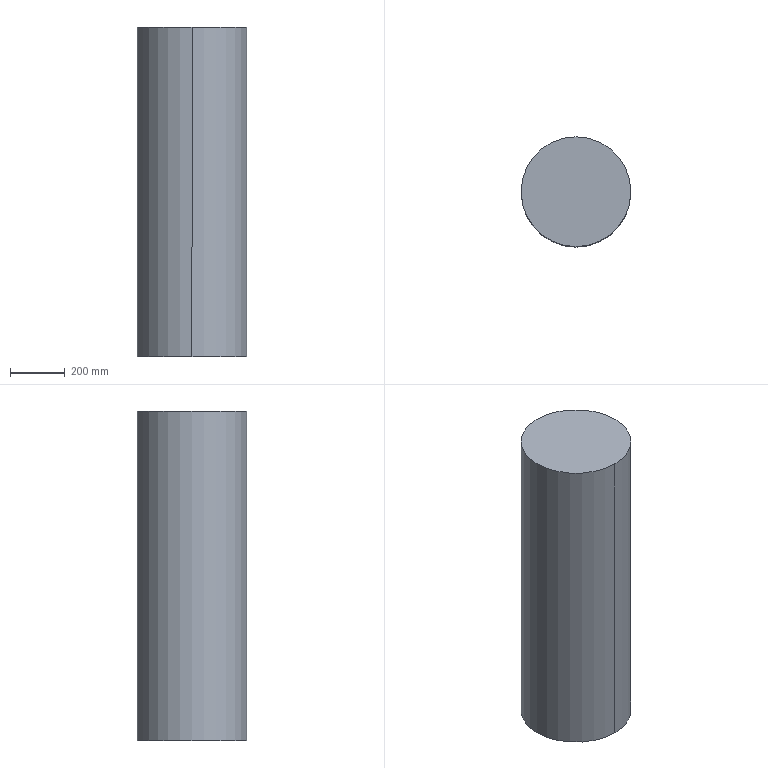Component | SolidWorks | FlexibleLegPinAxis-1 | 1 solid | 4 faces | box 400 x 400 x 1200 mm | volume 150796447 mm3 | cylinder 2 | plane 2 | commonest cylinder face diameters 400 x2
build123d program:
from build123d import *

# Parameters (mm, degrees)
SKETCH1_R           = 200
BOSS_EXTRUDE1_DEPTH = 1200


with BuildPart() as part:
    # Sketch1 → Boss-Extrude1 (new body)
    with BuildSketch(Plane(origin=(0, 0, 0), x_dir=(1, 0, 0), z_dir=(0, 1, 0))):
        with Locations(Location((0, 0, 0), (0, 0, 270))):
            Circle(SKETCH1_R)
    extrude(amount=BOSS_EXTRUDE1_DEPTH)


solid = part.part

# Placed as in the assembly
solid = solid.moved(Location((-4068.967, 20198.918, -12526.996), (90, 0, 0)))
STEP:
#1=COLOUR_RGB('',0.7922,0.8196,0.9333);
#2=FILL_AREA_STYLE_COLOUR('',#1);
#3=FILL_AREA_STYLE('',(#2));
#4=SURFACE_STYLE_FILL_AREA(#3);
#5=SURFACE_SIDE_STYLE('',(#4));
#6=SURFACE_STYLE_USAGE(.BOTH.,#5);
#7=PRESENTATION_STYLE_ASSIGNMENT((#6));
#8=CARTESIAN_POINT('',(-160.196,803.107,-493.189));
#9=VERTEX_POINT('',#8);
#10=CARTESIAN_POINT('',(-160.196,787.359,-493.189));
#11=VERTEX_POINT('',#10);
#12=CARTESIAN_POINT('',(-160.196,795.233,-493.189));
#13=DIRECTION('',(-0.0000002,0.,-1.));
#14=DIRECTION('',(-0.0000002,1.,0.));
#15=AXIS2_PLACEMENT_3D('',#12,#13,#14);
#16=CIRCLE('',#15,7.874);
#17=EDGE_CURVE('',#9,#11,#16,.T.);
#18=ORIENTED_EDGE('',*,*,#17,.F.);
#19=CARTESIAN_POINT('',(-160.196,803.107,-445.945));
#20=VERTEX_POINT('',#19);
#21=CARTESIAN_POINT('',(-160.196,803.107,-493.189));
#22=DIRECTION('',(0.0000002,-0.,1.));
#23=VECTOR('',#22,39.37);
#24=LINE('',#21,#23);
#25=EDGE_CURVE('',#9,#20,#24,.T.);
#26=ORIENTED_EDGE('',*,*,#25,.T.);
#27=CARTESIAN_POINT('',(-160.196,787.359,-445.945));
#28=VERTEX_POINT('',#27);
#29=CARTESIAN_POINT('',(-160.196,795.233,-445.945));
#30=DIRECTION('',(-0.0000002,0.,-1.));
#31=DIRECTION('',(-0.0000002,1.,0.));
#32=AXIS2_PLACEMENT_3D('',#29,#30,#31);
#33=CIRCLE('',#32,7.874);
#34=EDGE_CURVE('',#20,#28,#33,.T.);
#35=ORIENTED_EDGE('',*,*,#34,.T.);
#36=CARTESIAN_POINT('',(-160.196,787.359,-493.189));
#37=DIRECTION('',(0.0000002,-0.,1.));
#38=VECTOR('',#37,39.37);
#39=LINE('',#36,#38);
#40=EDGE_CURVE('',#11,#28,#39,.T.);
#41=ORIENTED_EDGE('',*,*,#40,.F.);
#42=EDGE_LOOP('',(#18,#26,#35,#41));
#43=FACE_OUTER_BOUND('',#42,.T.);
#44=CARTESIAN_POINT('',(-160.196,795.233,-493.189));
#45=DIRECTION('',(0.0000002,-0.,1.));
#46=DIRECTION('',(0.0000002,-1.,-0.));
#47=AXIS2_PLACEMENT_3D('',#44,#45,#46);
#48=CYLINDRICAL_SURFACE('',#47,7.874);
#49=ADVANCED_FACE('',(#43),#48,.T.);
#50=ORIENTED_EDGE('',*,*,#25,.F.);
#51=CARTESIAN_POINT('',(-160.196,795.233,-493.189));
#52=DIRECTION('',(-0.0000002,0.,-1.));
#53=DIRECTION('',(-0.0000002,1.,0.));
#54=AXIS2_PLACEMENT_3D('',#51,#52,#53);
#55=CIRCLE('',#54,7.874);
#56=EDGE_CURVE('',#11,#9,#55,.T.);
#57=ORIENTED_EDGE('',*,*,#56,.F.);
#58=ORIENTED_EDGE('',*,*,#40,.T.);
#59=CARTESIAN_POINT('',(-160.196,795.233,-445.945));
#60=DIRECTION('',(-0.0000002,0.,-1.));
#61=DIRECTION('',(-0.0000002,1.,0.));
#62=AXIS2_PLACEMENT_3D('',#59,#60,#61);
#63=CIRCLE('',#62,7.874);
#64=EDGE_CURVE('',#28,#20,#63,.T.);
#65=ORIENTED_EDGE('',*,*,#64,.T.);
#66=EDGE_LOOP('',(#50,#57,#58,#65));
#67=FACE_OUTER_BOUND('',#66,.T.);
#68=CARTESIAN_POINT('',(-160.196,795.233,-493.189));
#69=DIRECTION('',(0.0000002,-0.,1.));
#70=DIRECTION('',(0.0000002,-1.,-0.));
#71=AXIS2_PLACEMENT_3D('',#68,#69,#70);
#72=CYLINDRICAL_SURFACE('',#71,7.874);
#73=ADVANCED_FACE('',(#67),#72,.T.);
#74=ORIENTED_EDGE('',*,*,#56,.T.);
#75=ORIENTED_EDGE('',*,*,#17,.T.);
#76=EDGE_LOOP('',(#74,#75));
#77=FACE_OUTER_BOUND('',#76,.T.);
#78=CARTESIAN_POINT('',(-160.196,795.233,-493.189));
#79=DIRECTION('',(-0.0000002,0.,-1.));
#80=DIRECTION('',(-0.0000002,1.,0.));
#81=AXIS2_PLACEMENT_3D('',#78,#79,#80);
#82=PLANE('',#81);
#83=ADVANCED_FACE('',(#77),#82,.T.);
#84=ORIENTED_EDGE('',*,*,#64,.F.);
#85=ORIENTED_EDGE('',*,*,#34,.F.);
#86=EDGE_LOOP('',(#84,#85));
#87=FACE_OUTER_BOUND('',#86,.T.);
#88=CARTESIAN_POINT('',(-160.196,795.233,-445.945));
#89=DIRECTION('',(-0.0000002,0.,-1.));
#90=DIRECTION('',(-0.0000002,1.,0.));
#91=AXIS2_PLACEMENT_3D('',#88,#89,#90);
#92=PLANE('',#91);
#93=ADVANCED_FACE('',(#87),#92,.F.);
#94=CLOSED_SHELL('',(#49,#73,#83,#93));
#95=MANIFOLD_SOLID_BREP('',#94);
#96=STYLED_ITEM('',(#7),#95);
#97=PRESENTATION_LAYER_ASSIGNMENT('','',(#96));
#98=(LENGTH_UNIT()NAMED_UNIT(*)SI_UNIT($,.METRE.));
#99=LENGTH_MEASURE_WITH_UNIT(LENGTH_MEASURE(0.0254),#98);
#100=DIMENSIONAL_EXPONENTS(1.,0.,0.,0.,0.,0.,0.);
#101=(CONVERSION_BASED_UNIT('',#99)LENGTH_UNIT()NAMED_UNIT(#100));
#102=UNCERTAINTY_MEASURE_WITH_UNIT(LENGTH_MEASURE(0.00001),#101,'','');
#103=(NAMED_UNIT(*)PLANE_ANGLE_UNIT()SI_UNIT($,.RADIAN.));
#104=(NAMED_UNIT(*)SI_UNIT($,.STERADIAN.)SOLID_ANGLE_UNIT());
#105=(GEOMETRIC_REPRESENTATION_CONTEXT(3)GLOBAL_UNCERTAINTY_ASSIGNED_CONTEXT((#102))GLOBAL_UNIT_ASSIGNED_CONTEXT((#101,#103,#104))REPRESENTATION_CONTEXT('',''));
#106=MECHANICAL_DESIGN_GEOMETRIC_PRESENTATION_REPRESENTATION('',(#96),#105);
#107=CARTESIAN_POINT('',(0.,0.,0.));
#108=DIRECTION('',(0.,0.,1.));
#109=DIRECTION('',(1.,0.,0.));
#110=AXIS2_PLACEMENT_3D('',#107,#108,#109);
#111=(LENGTH_UNIT()NAMED_UNIT(*)SI_UNIT($,.METRE.));
#112=LENGTH_MEASURE_WITH_UNIT(LENGTH_MEASURE(0.0254),#111);
#113=DIMENSIONAL_EXPONENTS(1.,0.,0.,0.,0.,0.,0.);
#114=(CONVERSION_BASED_UNIT('',#112)LENGTH_UNIT()NAMED_UNIT(#113));
#115=UNCERTAINTY_MEASURE_WITH_UNIT(LENGTH_MEASURE(0.00001),#114,'','');
#116=(NAMED_UNIT(*)PLANE_ANGLE_UNIT()SI_UNIT($,.RADIAN.));
#117=(NAMED_UNIT(*)SI_UNIT($,.STERADIAN.)SOLID_ANGLE_UNIT());
#118=(GEOMETRIC_REPRESENTATION_CONTEXT(3)GLOBAL_UNCERTAINTY_ASSIGNED_CONTEXT((#115))GLOBAL_UNIT_ASSIGNED_CONTEXT((#114,#116,#117))REPRESENTATION_CONTEXT('',''));
#119=ADVANCED_BREP_SHAPE_REPRESENTATION('',(#95,#110),#118);